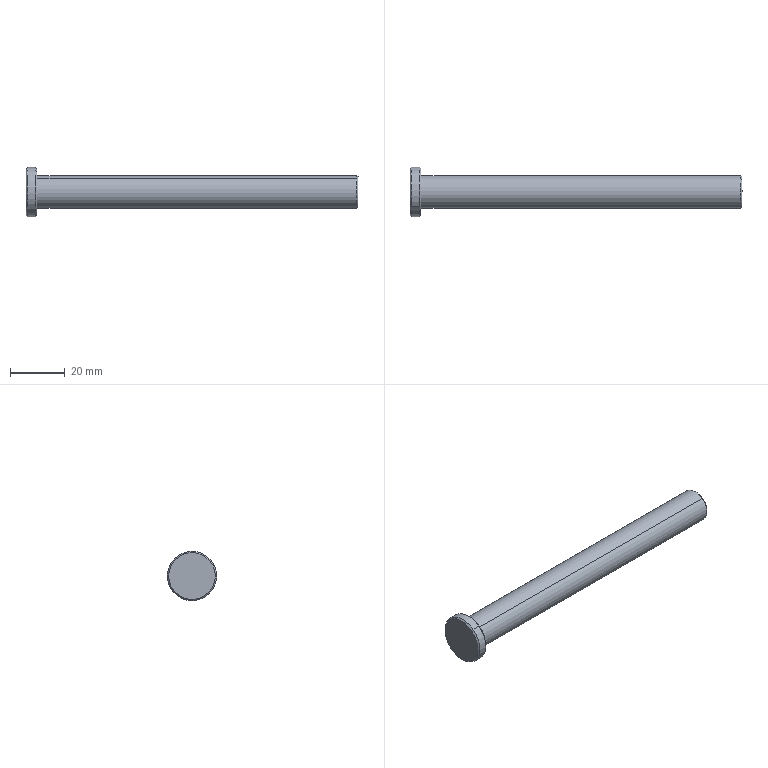Component | SolidWorks | TieRod-1 | 1 solid | 17 faces | box 121 x 18 x 18 mm | volume 13399 mm3 | cone 8 | cylinder 6 | plane 3 | commonest cylinder face diameters 6.8 x2 18 x2 12 x2
build123d program:
from build123d import *

# Parameters (mm, degrees)
SKETCH1_R             = 6
BOSS_EXTRUDE1_DEPTH   = 117
SKETCH2_R             = 9
BOSS_EXTRUDE2_DEPTH   = 4
M8_TAPPED_HOLE1_D     = 6.8
M8_TAPPED_HOLE1_DEPTH = 22.25
M8_TAPPED_HOLE1_TIP   = 2.043
CHAMFER1_SIZE         = 0.5


with BuildPart() as part:
    # Sketch1 → Boss-Extrude1 (new body)
    with BuildSketch(Plane.XY):
        Circle(SKETCH1_R)
    extrude(amount=BOSS_EXTRUDE1_DEPTH)

    # Sketch2 → Boss-Extrude2 (add)
    with BuildSketch(Plane.XY.offset(117)):
        Circle(SKETCH2_R)
    extrude(amount=BOSS_EXTRUDE2_DEPTH)

    # M8 Tapped Hole1
    with Locations(Plane(origin=(0, 0, 0), x_dir=(-1, 0, 0), z_dir=(0, 0, -1))):
        with Locations((0, 0)):
            Hole(M8_TAPPED_HOLE1_D / 2, depth=M8_TAPPED_HOLE1_DEPTH)
            with Locations((0, 0, -(M8_TAPPED_HOLE1_DEPTH + M8_TAPPED_HOLE1_TIP / 2))):  # 118° drill point
                Cone(0, M8_TAPPED_HOLE1_D / 2, M8_TAPPED_HOLE1_TIP, mode=Mode.SUBTRACT)

    # Chamfer1
    chamfer1_edges = [part.edges().sort_by_distance(p)[0] for p in [
        (-6, 0, 0),
        (-9, 0, 117),
        (-9, 0, 121),
    ]]
    chamfer(chamfer1_edges, length=CHAMFER1_SIZE)


solid = part.part

# Placed as in the assembly
solid = solid.moved(Location((195.546, 42, 438.671), (0, -90, 0)))
STEP:
#1=COLOUR_RGB('',0.7922,0.8196,0.9333);
#2=FILL_AREA_STYLE_COLOUR('',#1);
#3=FILL_AREA_STYLE('',(#2));
#4=SURFACE_STYLE_FILL_AREA(#3);
#5=SURFACE_SIDE_STYLE('',(#4));
#6=SURFACE_STYLE_USAGE(.BOTH.,#5);
#7=PRESENTATION_STYLE_ASSIGNMENT((#6));
#8=CARTESIAN_POINT('',(3.092,1.453,17.538));
#9=VERTEX_POINT('',#8);
#10=CARTESIAN_POINT('',(3.092,1.854,17.003));
#11=VERTEX_POINT('',#10);
#12=CARTESIAN_POINT('',(3.092,1.654,17.271));
#13=DIRECTION('',(1.,0.,-0.));
#14=DIRECTION('',(-0.,0.5996,-0.8003));
#15=AXIS2_PLACEMENT_3D('',#12,#13,#14);
#16=CIRCLE('',#15,0.3346);
#17=EDGE_CURVE('',#9,#11,#16,.T.);
#18=ORIENTED_EDGE('',*,*,#17,.F.);
#19=CARTESIAN_POINT('',(3.073,1.441,17.554));
#20=VERTEX_POINT('',#19);
#21=CARTESIAN_POINT('',(3.073,1.441,17.554));
#22=DIRECTION('',(-0.7071,-0.424,0.5659));
#23=VECTOR('',#22,39.37);
#24=LINE('',#21,#23);
#25=EDGE_CURVE('',#9,#20,#24,.T.);
#26=ORIENTED_EDGE('',*,*,#25,.T.);
#27=CARTESIAN_POINT('',(3.073,1.866,16.987));
#28=VERTEX_POINT('',#27);
#29=CARTESIAN_POINT('',(3.073,1.654,17.271));
#30=DIRECTION('',(-1.,-0.,0.));
#31=DIRECTION('',(-0.,0.5996,-0.8003));
#32=AXIS2_PLACEMENT_3D('',#29,#30,#31);
#33=CIRCLE('',#32,0.3543);
#34=EDGE_CURVE('',#28,#20,#33,.T.);
#35=ORIENTED_EDGE('',*,*,#34,.F.);
#36=CARTESIAN_POINT('',(3.073,1.866,16.987));
#37=DIRECTION('',(-0.7071,0.424,-0.5659));
#38=VECTOR('',#37,39.37);
#39=LINE('',#36,#38);
#40=EDGE_CURVE('',#11,#28,#39,.T.);
#41=ORIENTED_EDGE('',*,*,#40,.F.);
#42=EDGE_LOOP('',(#18,#26,#35,#41));
#43=FACE_OUTER_BOUND('',#42,.T.);
#44=CARTESIAN_POINT('',(3.073,1.654,17.271));
#45=DIRECTION('',(-1.,-0.,0.));
#46=DIRECTION('',(-0.,0.5996,-0.8003));
#47=AXIS2_PLACEMENT_3D('',#44,#45,#46);
#48=CONICAL_SURFACE('',#47,0.3543,0.7854);
#49=ADVANCED_FACE('',(#43),#48,.T.);
#50=CARTESIAN_POINT('',(2.935,1.854,17.003));
#51=VERTEX_POINT('',#50);
#52=CARTESIAN_POINT('',(2.935,1.453,17.538));
#53=VERTEX_POINT('',#52);
#54=CARTESIAN_POINT('',(2.935,1.654,17.271));
#55=DIRECTION('',(-1.,-0.,0.));
#56=DIRECTION('',(-0.,0.5996,-0.8003));
#57=AXIS2_PLACEMENT_3D('',#54,#55,#56);
#58=CIRCLE('',#57,0.3346);
#59=EDGE_CURVE('',#51,#53,#58,.T.);
#60=ORIENTED_EDGE('',*,*,#59,.F.);
#61=CARTESIAN_POINT('',(2.955,1.866,16.987));
#62=VERTEX_POINT('',#61);
#63=CARTESIAN_POINT('',(2.935,1.854,17.003));
#64=DIRECTION('',(0.7071,0.424,-0.5659));
#65=VECTOR('',#64,39.37);
#66=LINE('',#63,#65);
#67=EDGE_CURVE('',#51,#62,#66,.T.);
#68=ORIENTED_EDGE('',*,*,#67,.T.);
#69=CARTESIAN_POINT('',(2.955,1.441,17.554));
#70=VERTEX_POINT('',#69);
#71=CARTESIAN_POINT('',(2.955,1.654,17.271));
#72=DIRECTION('',(1.,0.,-0.));
#73=DIRECTION('',(-0.,0.5996,-0.8003));
#74=AXIS2_PLACEMENT_3D('',#71,#72,#73);
#75=CIRCLE('',#74,0.3543);
#76=EDGE_CURVE('',#70,#62,#75,.T.);
#77=ORIENTED_EDGE('',*,*,#76,.F.);
#78=CARTESIAN_POINT('',(2.935,1.453,17.538));
#79=DIRECTION('',(0.7071,-0.424,0.5659));
#80=VECTOR('',#79,39.37);
#81=LINE('',#78,#80);
#82=EDGE_CURVE('',#53,#70,#81,.T.);
#83=ORIENTED_EDGE('',*,*,#82,.F.);
#84=EDGE_LOOP('',(#60,#68,#77,#83));
#85=FACE_OUTER_BOUND('',#84,.T.);
#86=CARTESIAN_POINT('',(2.935,1.654,17.271));
#87=DIRECTION('',(1.,0.,-0.));
#88=DIRECTION('',(0.,-0.5996,0.8003));
#89=AXIS2_PLACEMENT_3D('',#86,#87,#88);
#90=CONICAL_SURFACE('',#89,0.3346,0.7854);
#91=ADVANCED_FACE('',(#85),#90,.T.);
#92=CARTESIAN_POINT('',(7.699,1.524,17.444));
#93=VERTEX_POINT('',#92);
#94=CARTESIAN_POINT('',(7.699,1.783,17.097));
#95=VERTEX_POINT('',#94);
#96=CARTESIAN_POINT('',(7.699,1.654,17.271));
#97=DIRECTION('',(1.,0.,-0.));
#98=DIRECTION('',(-0.,0.5996,-0.8003));
#99=AXIS2_PLACEMENT_3D('',#96,#97,#98);
#100=CIRCLE('',#99,0.2165);
#101=EDGE_CURVE('',#93,#95,#100,.T.);
#102=ORIENTED_EDGE('',*,*,#101,.F.);
#103=CARTESIAN_POINT('',(7.679,1.512,17.46));
#104=VERTEX_POINT('',#103);
#105=CARTESIAN_POINT('',(7.679,1.512,17.46));
#106=DIRECTION('',(-0.7071,-0.424,0.5659));
#107=VECTOR('',#106,39.37);
#108=LINE('',#105,#107);
#109=EDGE_CURVE('',#93,#104,#108,.T.);
#110=ORIENTED_EDGE('',*,*,#109,.T.);
#111=CARTESIAN_POINT('',(7.679,1.795,17.081));
#112=VERTEX_POINT('',#111);
#113=CARTESIAN_POINT('',(7.679,1.654,17.271));
#114=DIRECTION('',(-1.,-0.,0.));
#115=DIRECTION('',(-0.,0.5996,-0.8003));
#116=AXIS2_PLACEMENT_3D('',#113,#114,#115);
#117=CIRCLE('',#116,0.2362);
#118=EDGE_CURVE('',#112,#104,#117,.T.);
#119=ORIENTED_EDGE('',*,*,#118,.F.);
#120=CARTESIAN_POINT('',(7.679,1.795,17.081));
#121=DIRECTION('',(-0.7071,0.424,-0.5659));
#122=VECTOR('',#121,39.37);
#123=LINE('',#120,#122);
#124=EDGE_CURVE('',#95,#112,#123,.T.);
#125=ORIENTED_EDGE('',*,*,#124,.F.);
#126=EDGE_LOOP('',(#102,#110,#119,#125));
#127=FACE_OUTER_BOUND('',#126,.T.);
#128=CARTESIAN_POINT('',(7.679,1.654,17.271));
#129=DIRECTION('',(-1.,-0.,0.));
#130=DIRECTION('',(-0.,0.5996,-0.8003));
#131=AXIS2_PLACEMENT_3D('',#128,#129,#130);
#132=CONICAL_SURFACE('',#131,0.2362,0.7854);
#133=ADVANCED_FACE('',(#127),#132,.T.);
#134=CARTESIAN_POINT('',(6.823,1.734,17.163));
#135=VERTEX_POINT('',#134);
#136=CARTESIAN_POINT('',(6.823,1.573,17.378));
#137=VERTEX_POINT('',#136);
#138=CARTESIAN_POINT('',(6.823,1.654,17.271));
#139=DIRECTION('',(1.,0.,-0.));
#140=DIRECTION('',(0.,-0.5996,0.8003));
#141=AXIS2_PLACEMENT_3D('',#138,#139,#140);
#142=CIRCLE('',#141,0.1339);
#143=EDGE_CURVE('',#135,#137,#142,.T.);
#144=ORIENTED_EDGE('',*,*,#143,.F.);
#145=CARTESIAN_POINT('',(7.699,1.734,17.163));
#146=VERTEX_POINT('',#145);
#147=CARTESIAN_POINT('',(7.699,1.734,17.163));
#148=DIRECTION('',(1.,0.,-0.));
#149=VECTOR('',#148,39.37);
#150=LINE('',#147,#149);
#151=EDGE_CURVE('',#135,#146,#150,.T.);
#152=ORIENTED_EDGE('',*,*,#151,.T.);
#153=CARTESIAN_POINT('',(7.699,1.573,17.378));
#154=VERTEX_POINT('',#153);
#155=CARTESIAN_POINT('',(7.699,1.654,17.271));
#156=DIRECTION('',(1.,0.,-0.));
#157=DIRECTION('',(0.,-0.5996,0.8003));
#158=AXIS2_PLACEMENT_3D('',#155,#156,#157);
#159=CIRCLE('',#158,0.1339);
#160=EDGE_CURVE('',#146,#154,#159,.T.);
#161=ORIENTED_EDGE('',*,*,#160,.T.);
#162=CARTESIAN_POINT('',(7.699,1.573,17.378));
#163=DIRECTION('',(1.,0.,-0.));
#164=VECTOR('',#163,39.37);
#165=LINE('',#162,#164);
#166=EDGE_CURVE('',#137,#154,#165,.T.);
#167=ORIENTED_EDGE('',*,*,#166,.F.);
#168=EDGE_LOOP('',(#144,#152,#161,#167));
#169=FACE_OUTER_BOUND('',#168,.T.);
#170=CARTESIAN_POINT('',(7.699,1.654,17.271));
#171=DIRECTION('',(1.,0.,-0.));
#172=DIRECTION('',(0.,-0.5996,0.8003));
#173=AXIS2_PLACEMENT_3D('',#170,#171,#172);
#174=CYLINDRICAL_SURFACE('',#173,0.1339);
#175=ADVANCED_FACE('',(#169),#174,.F.);
#176=CARTESIAN_POINT('',(6.742,1.654,17.271));
#177=VERTEX_POINT('',#176);
#178=CARTESIAN_POINT('',(6.823,1.573,17.378));
#179=DIRECTION('',(0.515,-0.5139,0.686));
#180=VECTOR('',#179,39.37);
#181=LINE('',#178,#180);
#182=EDGE_CURVE('',#177,#137,#181,.T.);
#183=ORIENTED_EDGE('',*,*,#182,.F.);
#184=CARTESIAN_POINT('',(6.823,1.734,17.163));
#185=DIRECTION('',(0.515,0.5139,-0.686));
#186=VECTOR('',#185,39.37);
#187=LINE('',#184,#186);
#188=EDGE_CURVE('',#177,#135,#187,.T.);
#189=ORIENTED_EDGE('',*,*,#188,.T.);
#190=ORIENTED_EDGE('',*,*,#143,.T.);
#191=EDGE_LOOP('',(#183,#189,#190));
#192=FACE_OUTER_BOUND('',#191,.T.);
#193=CARTESIAN_POINT('',(6.823,1.654,17.271));
#194=DIRECTION('',(1.,0.,-0.));
#195=DIRECTION('',(0.,-0.5996,0.8003));
#196=AXIS2_PLACEMENT_3D('',#193,#194,#195);
#197=CONICAL_SURFACE('',#196,0.1339,1.03);
#198=ADVANCED_FACE('',(#192),#197,.F.);
#199=ORIENTED_EDGE('',*,*,#76,.T.);
#200=CARTESIAN_POINT('',(2.935,1.866,16.987));
#201=DIRECTION('',(1.,0.,-0.));
#202=VECTOR('',#201,39.37);
#203=LINE('',#200,#202);
#204=EDGE_CURVE('',#62,#28,#203,.T.);
#205=ORIENTED_EDGE('',*,*,#204,.T.);
#206=ORIENTED_EDGE('',*,*,#34,.T.);
#207=CARTESIAN_POINT('',(2.935,1.441,17.554));
#208=DIRECTION('',(1.,0.,-0.));
#209=VECTOR('',#208,39.37);
#210=LINE('',#207,#209);
#211=EDGE_CURVE('',#70,#20,#210,.T.);
#212=ORIENTED_EDGE('',*,*,#211,.F.);
#213=EDGE_LOOP('',(#199,#205,#206,#212));
#214=FACE_OUTER_BOUND('',#213,.T.);
#215=CARTESIAN_POINT('',(2.935,1.654,17.271));
#216=DIRECTION('',(1.,0.,-0.));
#217=DIRECTION('',(0.,-0.5996,0.8003));
#218=AXIS2_PLACEMENT_3D('',#215,#216,#217);
#219=CYLINDRICAL_SURFACE('',#218,0.3543);
#220=ADVANCED_FACE('',(#214),#219,.T.);
#221=CARTESIAN_POINT('',(3.092,1.795,17.081));
#222=VERTEX_POINT('',#221);
#223=CARTESIAN_POINT('',(3.092,1.512,17.46));
#224=VERTEX_POINT('',#223);
#225=CARTESIAN_POINT('',(3.092,1.654,17.271));
#226=DIRECTION('',(-1.,-0.,0.));
#227=DIRECTION('',(-0.,0.5996,-0.8003));
#228=AXIS2_PLACEMENT_3D('',#225,#226,#227);
#229=CIRCLE('',#228,0.2362);
#230=EDGE_CURVE('',#222,#224,#229,.T.);
#231=ORIENTED_EDGE('',*,*,#230,.F.);
#232=CARTESIAN_POINT('',(3.092,1.795,17.081));
#233=DIRECTION('',(1.,0.,-0.));
#234=VECTOR('',#233,39.37);
#235=LINE('',#232,#234);
#236=EDGE_CURVE('',#222,#112,#235,.T.);
#237=ORIENTED_EDGE('',*,*,#236,.T.);
#238=ORIENTED_EDGE('',*,*,#118,.T.);
#239=CARTESIAN_POINT('',(3.092,1.512,17.46));
#240=DIRECTION('',(1.,0.,-0.));
#241=VECTOR('',#240,39.37);
#242=LINE('',#239,#241);
#243=EDGE_CURVE('',#224,#104,#242,.T.);
#244=ORIENTED_EDGE('',*,*,#243,.F.);
#245=EDGE_LOOP('',(#231,#237,#238,#244));
#246=FACE_OUTER_BOUND('',#245,.T.);
#247=CARTESIAN_POINT('',(3.092,1.654,17.271));
#248=DIRECTION('',(1.,0.,-0.));
#249=DIRECTION('',(0.,-0.5996,0.8003));
#250=AXIS2_PLACEMENT_3D('',#247,#248,#249);
#251=CYLINDRICAL_SURFACE('',#250,0.2362);
#252=ADVANCED_FACE('',(#246),#251,.T.);
#253=ORIENTED_EDGE('',*,*,#236,.F.);
#254=CARTESIAN_POINT('',(3.092,1.654,17.271));
#255=DIRECTION('',(-1.,-0.,0.));
#256=DIRECTION('',(-0.,0.5996,-0.8003));
#257=AXIS2_PLACEMENT_3D('',#254,#255,#256);
#258=CIRCLE('',#257,0.2362);
#259=EDGE_CURVE('',#224,#222,#258,.T.);
#260=ORIENTED_EDGE('',*,*,#259,.F.);
#261=ORIENTED_EDGE('',*,*,#243,.T.);
#262=CARTESIAN_POINT('',(7.679,1.654,17.271));
#263=DIRECTION('',(-1.,-0.,0.));
#264=DIRECTION('',(-0.,0.5996,-0.8003));
#265=AXIS2_PLACEMENT_3D('',#262,#263,#264);
#266=CIRCLE('',#265,0.2362);
#267=EDGE_CURVE('',#104,#112,#266,.T.);
#268=ORIENTED_EDGE('',*,*,#267,.T.);
#269=EDGE_LOOP('',(#253,#260,#261,#268));
#270=FACE_OUTER_BOUND('',#269,.T.);
#271=CARTESIAN_POINT('',(3.092,1.654,17.271));
#272=DIRECTION('',(1.,0.,-0.));
#273=DIRECTION('',(0.,-0.5996,0.8003));
#274=AXIS2_PLACEMENT_3D('',#271,#272,#273);
#275=CYLINDRICAL_SURFACE('',#274,0.2362);
#276=ADVANCED_FACE('',(#270),#275,.T.);
#277=CARTESIAN_POINT('',(7.699,1.654,17.271));
#278=DIRECTION('',(1.,0.,-0.));
#279=DIRECTION('',(-0.,0.5996,-0.8003));
#280=AXIS2_PLACEMENT_3D('',#277,#278,#279);
#281=CIRCLE('',#280,0.2165);
#282=EDGE_CURVE('',#95,#93,#281,.T.);
#283=ORIENTED_EDGE('',*,*,#282,.T.);
#284=ORIENTED_EDGE('',*,*,#101,.T.);
#285=EDGE_LOOP('',(#283,#284));
#286=FACE_OUTER_BOUND('',#285,.T.);
#287=CARTESIAN_POINT('',(7.699,1.654,17.271));
#288=DIRECTION('',(1.,0.,-0.));
#289=DIRECTION('',(0.,-0.5996,0.8003));
#290=AXIS2_PLACEMENT_3D('',#287,#288,#289);
#291=CIRCLE('',#290,0.1339);
#292=EDGE_CURVE('',#154,#146,#291,.T.);
#293=ORIENTED_EDGE('',*,*,#292,.F.);
#294=ORIENTED_EDGE('',*,*,#160,.F.);
#295=EDGE_LOOP('',(#293,#294));
#296=FACE_BOUND('',#295,.T.);
#297=CARTESIAN_POINT('',(7.699,1.654,17.271));
#298=DIRECTION('',(-1.,-0.,0.));
#299=DIRECTION('',(-0.,0.5996,-0.8003));
#300=AXIS2_PLACEMENT_3D('',#297,#298,#299);
#301=PLANE('',#300);
#302=ADVANCED_FACE('',(#286,#296),#301,.F.);
#303=ORIENTED_EDGE('',*,*,#204,.F.);
#304=CARTESIAN_POINT('',(2.955,1.654,17.271));
#305=DIRECTION('',(1.,0.,-0.));
#306=DIRECTION('',(-0.,0.5996,-0.8003));
#307=AXIS2_PLACEMENT_3D('',#304,#305,#306);
#308=CIRCLE('',#307,0.3543);
#309=EDGE_CURVE('',#62,#70,#308,.T.);
#310=ORIENTED_EDGE('',*,*,#309,.T.);
#311=ORIENTED_EDGE('',*,*,#211,.T.);
#312=CARTESIAN_POINT('',(3.073,1.654,17.271));
#313=DIRECTION('',(-1.,-0.,0.));
#314=DIRECTION('',(-0.,0.5996,-0.8003));
#315=AXIS2_PLACEMENT_3D('',#312,#313,#314);
#316=CIRCLE('',#315,0.3543);
#317=EDGE_CURVE('',#20,#28,#316,.T.);
#318=ORIENTED_EDGE('',*,*,#317,.T.);
#319=EDGE_LOOP('',(#303,#310,#311,#318));
#320=FACE_OUTER_BOUND('',#319,.T.);
#321=CARTESIAN_POINT('',(2.935,1.654,17.271));
#322=DIRECTION('',(1.,0.,-0.));
#323=DIRECTION('',(0.,-0.5996,0.8003));
#324=AXIS2_PLACEMENT_3D('',#321,#322,#323);
#325=CYLINDRICAL_SURFACE('',#324,0.3543);
#326=ADVANCED_FACE('',(#320),#325,.T.);
#327=CARTESIAN_POINT('',(2.935,1.654,17.271));
#328=DIRECTION('',(-1.,-0.,0.));
#329=DIRECTION('',(-0.,0.5996,-0.8003));
#330=AXIS2_PLACEMENT_3D('',#327,#328,#329);
#331=CIRCLE('',#330,0.3346);
#332=EDGE_CURVE('',#53,#51,#331,.T.);
#333=ORIENTED_EDGE('',*,*,#332,.T.);
#334=ORIENTED_EDGE('',*,*,#59,.T.);
#335=EDGE_LOOP('',(#333,#334));
#336=FACE_OUTER_BOUND('',#335,.T.);
#337=CARTESIAN_POINT('',(2.935,1.654,17.271));
#338=DIRECTION('',(-1.,-0.,0.));
#339=DIRECTION('',(-0.,0.5996,-0.8003));
#340=AXIS2_PLACEMENT_3D('',#337,#338,#339);
#341=PLANE('',#340);
#342=ADVANCED_FACE('',(#336),#341,.T.);
#343=CARTESIAN_POINT('',(3.092,1.654,17.271));
#344=DIRECTION('',(1.,0.,-0.));
#345=DIRECTION('',(-0.,0.5996,-0.8003));
#346=AXIS2_PLACEMENT_3D('',#343,#344,#345);
#347=CIRCLE('',#346,0.3346);
#348=EDGE_CURVE('',#11,#9,#347,.T.);
#349=ORIENTED_EDGE('',*,*,#348,.T.);
#350=ORIENTED_EDGE('',*,*,#17,.T.);
#351=EDGE_LOOP('',(#349,#350));
#352=FACE_OUTER_BOUND('',#351,.T.);
#353=ORIENTED_EDGE('',*,*,#259,.T.);
#354=ORIENTED_EDGE('',*,*,#230,.T.);
#355=EDGE_LOOP('',(#353,#354));
#356=FACE_BOUND('',#355,.T.);
#357=CARTESIAN_POINT('',(3.092,1.654,17.271));
#358=DIRECTION('',(-1.,-0.,0.));
#359=DIRECTION('',(-0.,0.5996,-0.8003));
#360=AXIS2_PLACEMENT_3D('',#357,#358,#359);
#361=PLANE('',#360);
#362=ADVANCED_FACE('',(#352,#356),#361,.F.);
#363=ORIENTED_EDGE('',*,*,#188,.F.);
#364=ORIENTED_EDGE('',*,*,#182,.T.);
#365=CARTESIAN_POINT('',(6.823,1.654,17.271));
#366=DIRECTION('',(1.,0.,-0.));
#367=DIRECTION('',(0.,-0.5996,0.8003));
#368=AXIS2_PLACEMENT_3D('',#365,#366,#367);
#369=CIRCLE('',#368,0.1339);
#370=EDGE_CURVE('',#137,#135,#369,.T.);
#371=ORIENTED_EDGE('',*,*,#370,.T.);
#372=EDGE_LOOP('',(#363,#364,#371));
#373=FACE_OUTER_BOUND('',#372,.T.);
#374=CARTESIAN_POINT('',(6.823,1.654,17.271));
#375=DIRECTION('',(1.,0.,-0.));
#376=DIRECTION('',(0.,-0.5996,0.8003));
#377=AXIS2_PLACEMENT_3D('',#374,#375,#376);
#378=CONICAL_SURFACE('',#377,0.1339,1.03);
#379=ADVANCED_FACE('',(#373),#378,.F.);
#380=ORIENTED_EDGE('',*,*,#151,.F.);
#381=ORIENTED_EDGE('',*,*,#370,.F.);
#382=ORIENTED_EDGE('',*,*,#166,.T.);
#383=ORIENTED_EDGE('',*,*,#292,.T.);
#384=EDGE_LOOP('',(#380,#381,#382,#383));
#385=FACE_OUTER_BOUND('',#384,.T.);
#386=CARTESIAN_POINT('',(7.699,1.654,17.271));
#387=DIRECTION('',(1.,0.,-0.));
#388=DIRECTION('',(0.,-0.5996,0.8003));
#389=AXIS2_PLACEMENT_3D('',#386,#387,#388);
#390=CYLINDRICAL_SURFACE('',#389,0.1339);
#391=ADVANCED_FACE('',(#385),#390,.F.);
#392=ORIENTED_EDGE('',*,*,#109,.F.);
#393=ORIENTED_EDGE('',*,*,#282,.F.);
#394=ORIENTED_EDGE('',*,*,#124,.T.);
#395=ORIENTED_EDGE('',*,*,#267,.F.);
#396=EDGE_LOOP('',(#392,#393,#394,#395));
#397=FACE_OUTER_BOUND('',#396,.T.);
#398=CARTESIAN_POINT('',(7.679,1.654,17.271));
#399=DIRECTION('',(-1.,-0.,0.));
#400=DIRECTION('',(-0.,0.5996,-0.8003));
#401=AXIS2_PLACEMENT_3D('',#398,#399,#400);
#402=CONICAL_SURFACE('',#401,0.2362,0.7854);
#403=ADVANCED_FACE('',(#397),#402,.T.);
#404=ORIENTED_EDGE('',*,*,#67,.F.);
#405=ORIENTED_EDGE('',*,*,#332,.F.);
#406=ORIENTED_EDGE('',*,*,#82,.T.);
#407=ORIENTED_EDGE('',*,*,#309,.F.);
#408=EDGE_LOOP('',(#404,#405,#406,#407));
#409=FACE_OUTER_BOUND('',#408,.T.);
#410=CARTESIAN_POINT('',(2.935,1.654,17.271));
#411=DIRECTION('',(1.,0.,-0.));
#412=DIRECTION('',(0.,-0.5996,0.8003));
#413=AXIS2_PLACEMENT_3D('',#410,#411,#412);
#414=CONICAL_SURFACE('',#413,0.3346,0.7854);
#415=ADVANCED_FACE('',(#409),#414,.T.);
#416=ORIENTED_EDGE('',*,*,#25,.F.);
#417=ORIENTED_EDGE('',*,*,#348,.F.);
#418=ORIENTED_EDGE('',*,*,#40,.T.);
#419=ORIENTED_EDGE('',*,*,#317,.F.);
#420=EDGE_LOOP('',(#416,#417,#418,#419));
#421=FACE_OUTER_BOUND('',#420,.T.);
#422=CARTESIAN_POINT('',(3.073,1.654,17.271));
#423=DIRECTION('',(-1.,-0.,0.));
#424=DIRECTION('',(-0.,0.5996,-0.8003));
#425=AXIS2_PLACEMENT_3D('',#422,#423,#424);
#426=CONICAL_SURFACE('',#425,0.3543,0.7854);
#427=ADVANCED_FACE('',(#421),#426,.T.);
#428=CLOSED_SHELL('',(#49,#91,#133,#175,#198,#220,#252,#276,#302,#326,#342,#362,#379,#391,#403,#415,#427));
#429=MANIFOLD_SOLID_BREP('',#428);
#430=STYLED_ITEM('',(#7),#429);
#431=(LENGTH_UNIT()NAMED_UNIT(*)SI_UNIT($,.METRE.));
#432=LENGTH_MEASURE_WITH_UNIT(LENGTH_MEASURE(0.0254),#431);
#433=DIMENSIONAL_EXPONENTS(1.,0.,0.,0.,0.,0.,0.);
#434=(CONVERSION_BASED_UNIT('',#432)LENGTH_UNIT()NAMED_UNIT(#433));
#435=UNCERTAINTY_MEASURE_WITH_UNIT(LENGTH_MEASURE(0.00001),#434,'','');
#436=(NAMED_UNIT(*)PLANE_ANGLE_UNIT()SI_UNIT($,.RADIAN.));
#437=(NAMED_UNIT(*)SI_UNIT($,.STERADIAN.)SOLID_ANGLE_UNIT());
#438=(GEOMETRIC_REPRESENTATION_CONTEXT(3)GLOBAL_UNCERTAINTY_ASSIGNED_CONTEXT((#435))GLOBAL_UNIT_ASSIGNED_CONTEXT((#434,#436,#437))REPRESENTATION_CONTEXT('',''));
#439=MECHANICAL_DESIGN_GEOMETRIC_PRESENTATION_REPRESENTATION('',(#430),#438);
#440=PRESENTATION_LAYER_ASSIGNMENT('','',(#430));
#441=CARTESIAN_POINT('',(0.,0.,0.));
#442=DIRECTION('',(0.,0.,1.));
#443=DIRECTION('',(1.,0.,0.));
#444=AXIS2_PLACEMENT_3D('',#441,#442,#443);
#445=(LENGTH_UNIT()NAMED_UNIT(*)SI_UNIT($,.METRE.));
#446=LENGTH_MEASURE_WITH_UNIT(LENGTH_MEASURE(0.0254),#445);
#447=DIMENSIONAL_EXPONENTS(1.,0.,0.,0.,0.,0.,0.);
#448=(CONVERSION_BASED_UNIT('',#446)LENGTH_UNIT()NAMED_UNIT(#447));
#449=UNCERTAINTY_MEASURE_WITH_UNIT(LENGTH_MEASURE(0.00001),#448,'','');
#450=(NAMED_UNIT(*)PLANE_ANGLE_UNIT()SI_UNIT($,.RADIAN.));
#451=(NAMED_UNIT(*)SI_UNIT($,.STERADIAN.)SOLID_ANGLE_UNIT());
#452=(GEOMETRIC_REPRESENTATION_CONTEXT(3)GLOBAL_UNCERTAINTY_ASSIGNED_CONTEXT((#449))GLOBAL_UNIT_ASSIGNED_CONTEXT((#448,#450,#451))REPRESENTATION_CONTEXT('',''));
#453=ADVANCED_BREP_SHAPE_REPRESENTATION('',(#429,#444),#452);